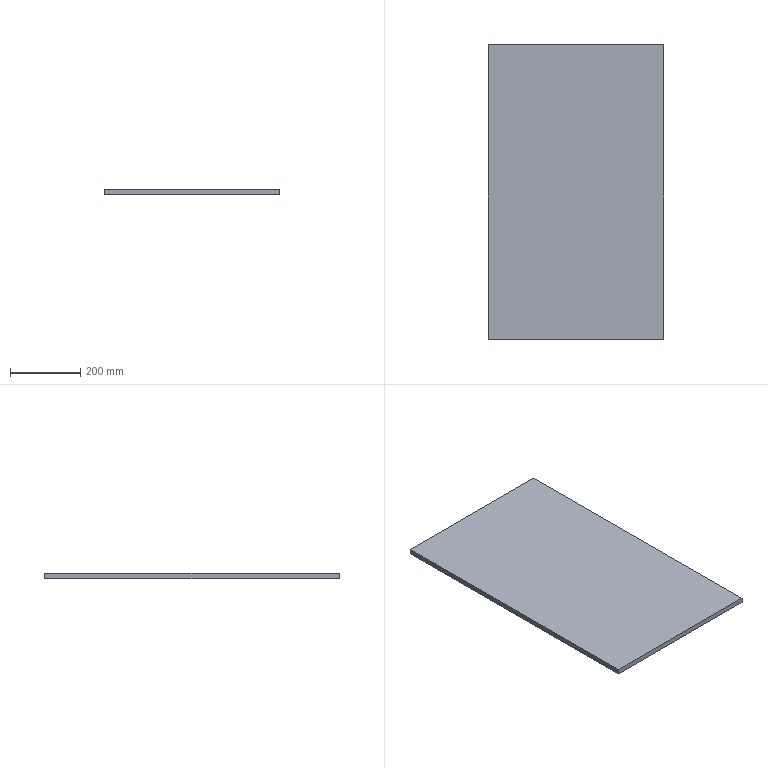Component | SolidWorks | FrameSupportPlate1122-1 | 1 solid | 6 faces | box 500 x 840 x 15 mm | volume 6300000 mm3 | plane 6
build123d program:
from build123d import *

# Parameters (mm, degrees)
SKETCH1_W           = 500
SKETCH1_H           = 840
BOSS_EXTRUDE1_DEPTH = 15


with BuildPart() as part:
    # Sketch1 → Boss-Extrude1 (new body)
    with BuildSketch(Plane.XY):
        Rectangle(SKETCH1_W, SKETCH1_H)
    extrude(amount=BOSS_EXTRUDE1_DEPTH)


solid = part.part

# Placed as in the assembly
solid = solid.moved(Location((-84.479, 144.741, 790), (0, 0, 0)))
STEP:
#1=COLOUR_RGB('',0.7922,0.8196,0.9333);
#2=FILL_AREA_STYLE_COLOUR('',#1);
#3=FILL_AREA_STYLE('',(#2));
#4=SURFACE_STYLE_FILL_AREA(#3);
#5=SURFACE_SIDE_STYLE('',(#4));
#6=SURFACE_STYLE_USAGE(.BOTH.,#5);
#7=PRESENTATION_STYLE_ASSIGNMENT((#6));
#8=CARTESIAN_POINT('',(6.517,-10.837,31.102));
#9=VERTEX_POINT('',#8);
#10=CARTESIAN_POINT('',(6.517,22.234,31.102));
#11=VERTEX_POINT('',#10);
#12=CARTESIAN_POINT('',(6.517,-10.837,31.102));
#13=DIRECTION('',(0.,1.,0.));
#14=VECTOR('',#13,39.37);
#15=LINE('',#12,#14);
#16=EDGE_CURVE('',#9,#11,#15,.T.);
#17=ORIENTED_EDGE('',*,*,#16,.T.);
#18=CARTESIAN_POINT('',(6.517,22.234,31.693));
#19=VERTEX_POINT('',#18);
#20=CARTESIAN_POINT('',(6.517,22.234,31.693));
#21=DIRECTION('',(0.,0.,-1.));
#22=VECTOR('',#21,39.37);
#23=LINE('',#20,#22);
#24=EDGE_CURVE('',#19,#11,#23,.T.);
#25=ORIENTED_EDGE('',*,*,#24,.F.);
#26=CARTESIAN_POINT('',(6.517,-10.837,31.693));
#27=VERTEX_POINT('',#26);
#28=CARTESIAN_POINT('',(6.517,-10.837,31.693));
#29=DIRECTION('',(0.,1.,0.));
#30=VECTOR('',#29,39.37);
#31=LINE('',#28,#30);
#32=EDGE_CURVE('',#27,#19,#31,.T.);
#33=ORIENTED_EDGE('',*,*,#32,.F.);
#34=CARTESIAN_POINT('',(6.517,-10.837,31.693));
#35=DIRECTION('',(0.,0.,-1.));
#36=VECTOR('',#35,39.37);
#37=LINE('',#34,#36);
#38=EDGE_CURVE('',#27,#9,#37,.T.);
#39=ORIENTED_EDGE('',*,*,#38,.T.);
#40=EDGE_LOOP('',(#17,#25,#33,#39));
#41=FACE_OUTER_BOUND('',#40,.T.);
#42=CARTESIAN_POINT('',(6.517,-10.837,31.693));
#43=DIRECTION('',(-1.,0.,0.));
#44=DIRECTION('',(0.,0.,1.));
#45=AXIS2_PLACEMENT_3D('',#42,#43,#44);
#46=PLANE('',#45);
#47=ADVANCED_FACE('',(#41),#46,.F.);
#48=CARTESIAN_POINT('',(-13.168,22.234,31.102));
#49=VERTEX_POINT('',#48);
#50=CARTESIAN_POINT('',(-13.168,22.234,31.102));
#51=DIRECTION('',(-1.,0.,0.));
#52=VECTOR('',#51,39.37);
#53=LINE('',#50,#52);
#54=EDGE_CURVE('',#11,#49,#53,.T.);
#55=ORIENTED_EDGE('',*,*,#54,.T.);
#56=CARTESIAN_POINT('',(-13.168,22.234,31.693));
#57=VERTEX_POINT('',#56);
#58=CARTESIAN_POINT('',(-13.168,22.234,31.693));
#59=DIRECTION('',(0.,0.,-1.));
#60=VECTOR('',#59,39.37);
#61=LINE('',#58,#60);
#62=EDGE_CURVE('',#57,#49,#61,.T.);
#63=ORIENTED_EDGE('',*,*,#62,.F.);
#64=CARTESIAN_POINT('',(-13.168,22.234,31.693));
#65=DIRECTION('',(-1.,0.,0.));
#66=VECTOR('',#65,39.37);
#67=LINE('',#64,#66);
#68=EDGE_CURVE('',#19,#57,#67,.T.);
#69=ORIENTED_EDGE('',*,*,#68,.F.);
#70=ORIENTED_EDGE('',*,*,#24,.T.);
#71=EDGE_LOOP('',(#55,#63,#69,#70));
#72=FACE_OUTER_BOUND('',#71,.T.);
#73=CARTESIAN_POINT('',(-13.168,22.234,31.693));
#74=DIRECTION('',(0.,-1.,0.));
#75=DIRECTION('',(0.,0.,-1.));
#76=AXIS2_PLACEMENT_3D('',#73,#74,#75);
#77=PLANE('',#76);
#78=ADVANCED_FACE('',(#72),#77,.F.);
#79=CARTESIAN_POINT('',(-13.168,-10.837,31.102));
#80=VERTEX_POINT('',#79);
#81=CARTESIAN_POINT('',(-13.168,-10.837,31.102));
#82=DIRECTION('',(0.,-1.,0.));
#83=VECTOR('',#82,39.37);
#84=LINE('',#81,#83);
#85=EDGE_CURVE('',#49,#80,#84,.T.);
#86=ORIENTED_EDGE('',*,*,#85,.T.);
#87=CARTESIAN_POINT('',(-13.168,-10.837,31.693));
#88=VERTEX_POINT('',#87);
#89=CARTESIAN_POINT('',(-13.168,-10.837,31.693));
#90=DIRECTION('',(0.,0.,-1.));
#91=VECTOR('',#90,39.37);
#92=LINE('',#89,#91);
#93=EDGE_CURVE('',#88,#80,#92,.T.);
#94=ORIENTED_EDGE('',*,*,#93,.F.);
#95=CARTESIAN_POINT('',(-13.168,-10.837,31.693));
#96=DIRECTION('',(0.,-1.,0.));
#97=VECTOR('',#96,39.37);
#98=LINE('',#95,#97);
#99=EDGE_CURVE('',#57,#88,#98,.T.);
#100=ORIENTED_EDGE('',*,*,#99,.F.);
#101=ORIENTED_EDGE('',*,*,#62,.T.);
#102=EDGE_LOOP('',(#86,#94,#100,#101));
#103=FACE_OUTER_BOUND('',#102,.T.);
#104=CARTESIAN_POINT('',(-13.168,-10.837,31.693));
#105=DIRECTION('',(1.,0.,0.));
#106=DIRECTION('',(0.,0.,-1.));
#107=AXIS2_PLACEMENT_3D('',#104,#105,#106);
#108=PLANE('',#107);
#109=ADVANCED_FACE('',(#103),#108,.F.);
#110=CARTESIAN_POINT('',(-13.168,-10.837,31.102));
#111=DIRECTION('',(1.,0.,0.));
#112=VECTOR('',#111,39.37);
#113=LINE('',#110,#112);
#114=EDGE_CURVE('',#80,#9,#113,.T.);
#115=ORIENTED_EDGE('',*,*,#114,.T.);
#116=ORIENTED_EDGE('',*,*,#38,.F.);
#117=CARTESIAN_POINT('',(-13.168,-10.837,31.693));
#118=DIRECTION('',(1.,0.,0.));
#119=VECTOR('',#118,39.37);
#120=LINE('',#117,#119);
#121=EDGE_CURVE('',#88,#27,#120,.T.);
#122=ORIENTED_EDGE('',*,*,#121,.F.);
#123=ORIENTED_EDGE('',*,*,#93,.T.);
#124=EDGE_LOOP('',(#115,#116,#122,#123));
#125=FACE_OUTER_BOUND('',#124,.T.);
#126=CARTESIAN_POINT('',(-13.168,-10.837,31.693));
#127=DIRECTION('',(0.,1.,0.));
#128=DIRECTION('',(0.,0.,1.));
#129=AXIS2_PLACEMENT_3D('',#126,#127,#128);
#130=PLANE('',#129);
#131=ADVANCED_FACE('',(#125),#130,.F.);
#132=ORIENTED_EDGE('',*,*,#32,.T.);
#133=ORIENTED_EDGE('',*,*,#68,.T.);
#134=ORIENTED_EDGE('',*,*,#99,.T.);
#135=ORIENTED_EDGE('',*,*,#121,.T.);
#136=EDGE_LOOP('',(#132,#133,#134,#135));
#137=FACE_OUTER_BOUND('',#136,.T.);
#138=CARTESIAN_POINT('',(-3.326,5.698,31.693));
#139=DIRECTION('',(0.,0.,-1.));
#140=DIRECTION('',(-1.,0.,0.));
#141=AXIS2_PLACEMENT_3D('',#138,#139,#140);
#142=PLANE('',#141);
#143=ADVANCED_FACE('',(#137),#142,.F.);
#144=ORIENTED_EDGE('',*,*,#16,.F.);
#145=ORIENTED_EDGE('',*,*,#114,.F.);
#146=ORIENTED_EDGE('',*,*,#85,.F.);
#147=ORIENTED_EDGE('',*,*,#54,.F.);
#148=EDGE_LOOP('',(#144,#145,#146,#147));
#149=FACE_OUTER_BOUND('',#148,.T.);
#150=CARTESIAN_POINT('',(-3.326,5.698,31.102));
#151=DIRECTION('',(0.,0.,-1.));
#152=DIRECTION('',(-1.,0.,0.));
#153=AXIS2_PLACEMENT_3D('',#150,#151,#152);
#154=PLANE('',#153);
#155=ADVANCED_FACE('',(#149),#154,.T.);
#156=CLOSED_SHELL('',(#47,#78,#109,#131,#143,#155));
#157=MANIFOLD_SOLID_BREP('',#156);
#158=STYLED_ITEM('',(#7),#157);
#159=PRESENTATION_LAYER_ASSIGNMENT('','',(#158));
#160=CARTESIAN_POINT('',(0.,0.,0.));
#161=DIRECTION('',(0.,0.,1.));
#162=DIRECTION('',(1.,0.,0.));
#163=AXIS2_PLACEMENT_3D('',#160,#161,#162);
#164=(LENGTH_UNIT()NAMED_UNIT(*)SI_UNIT($,.METRE.));
#165=LENGTH_MEASURE_WITH_UNIT(LENGTH_MEASURE(0.0254),#164);
#166=DIMENSIONAL_EXPONENTS(1.,0.,0.,0.,0.,0.,0.);
#167=(CONVERSION_BASED_UNIT('',#165)LENGTH_UNIT()NAMED_UNIT(#166));
#168=UNCERTAINTY_MEASURE_WITH_UNIT(LENGTH_MEASURE(0.00001),#167,'','');
#169=(NAMED_UNIT(*)PLANE_ANGLE_UNIT()SI_UNIT($,.RADIAN.));
#170=(NAMED_UNIT(*)SI_UNIT($,.STERADIAN.)SOLID_ANGLE_UNIT());
#171=(GEOMETRIC_REPRESENTATION_CONTEXT(3)GLOBAL_UNCERTAINTY_ASSIGNED_CONTEXT((#168))GLOBAL_UNIT_ASSIGNED_CONTEXT((#167,#169,#170))REPRESENTATION_CONTEXT('',''));
#172=ADVANCED_BREP_SHAPE_REPRESENTATION('',(#157,#163),#171);
#173=(LENGTH_UNIT()NAMED_UNIT(*)SI_UNIT($,.METRE.));
#174=LENGTH_MEASURE_WITH_UNIT(LENGTH_MEASURE(0.0254),#173);
#175=DIMENSIONAL_EXPONENTS(1.,0.,0.,0.,0.,0.,0.);
#176=(CONVERSION_BASED_UNIT('',#174)LENGTH_UNIT()NAMED_UNIT(#175));
#177=UNCERTAINTY_MEASURE_WITH_UNIT(LENGTH_MEASURE(0.00001),#176,'','');
#178=(NAMED_UNIT(*)PLANE_ANGLE_UNIT()SI_UNIT($,.RADIAN.));
#179=(NAMED_UNIT(*)SI_UNIT($,.STERADIAN.)SOLID_ANGLE_UNIT());
#180=(GEOMETRIC_REPRESENTATION_CONTEXT(3)GLOBAL_UNCERTAINTY_ASSIGNED_CONTEXT((#177))GLOBAL_UNIT_ASSIGNED_CONTEXT((#176,#178,#179))REPRESENTATION_CONTEXT('',''));
#181=MECHANICAL_DESIGN_GEOMETRIC_PRESENTATION_REPRESENTATION('',(#158),#180);